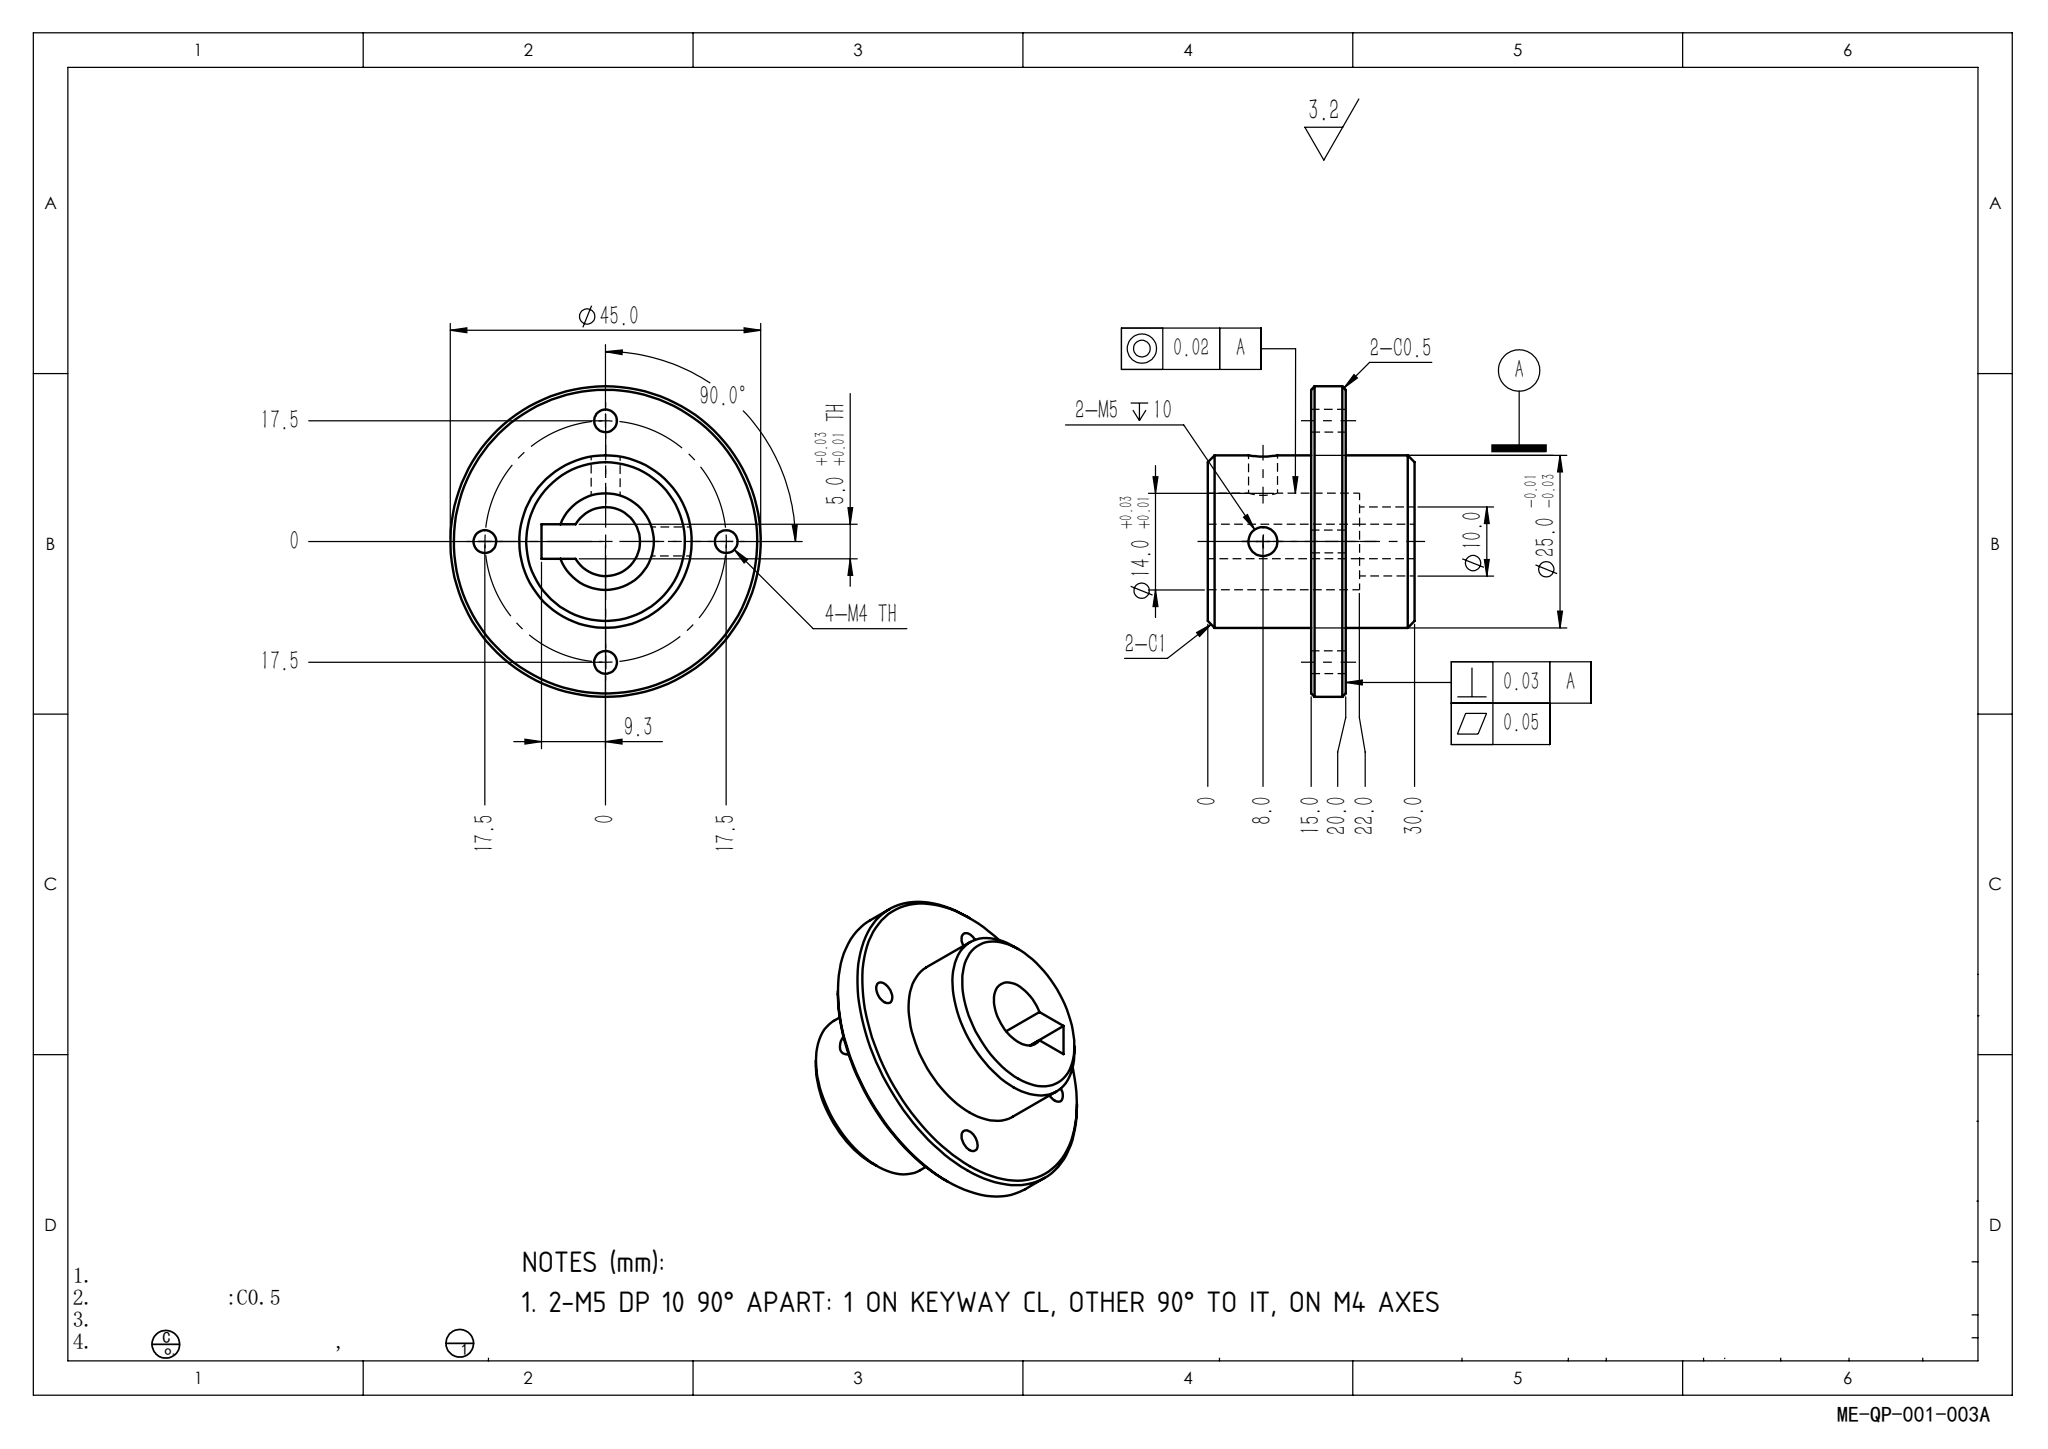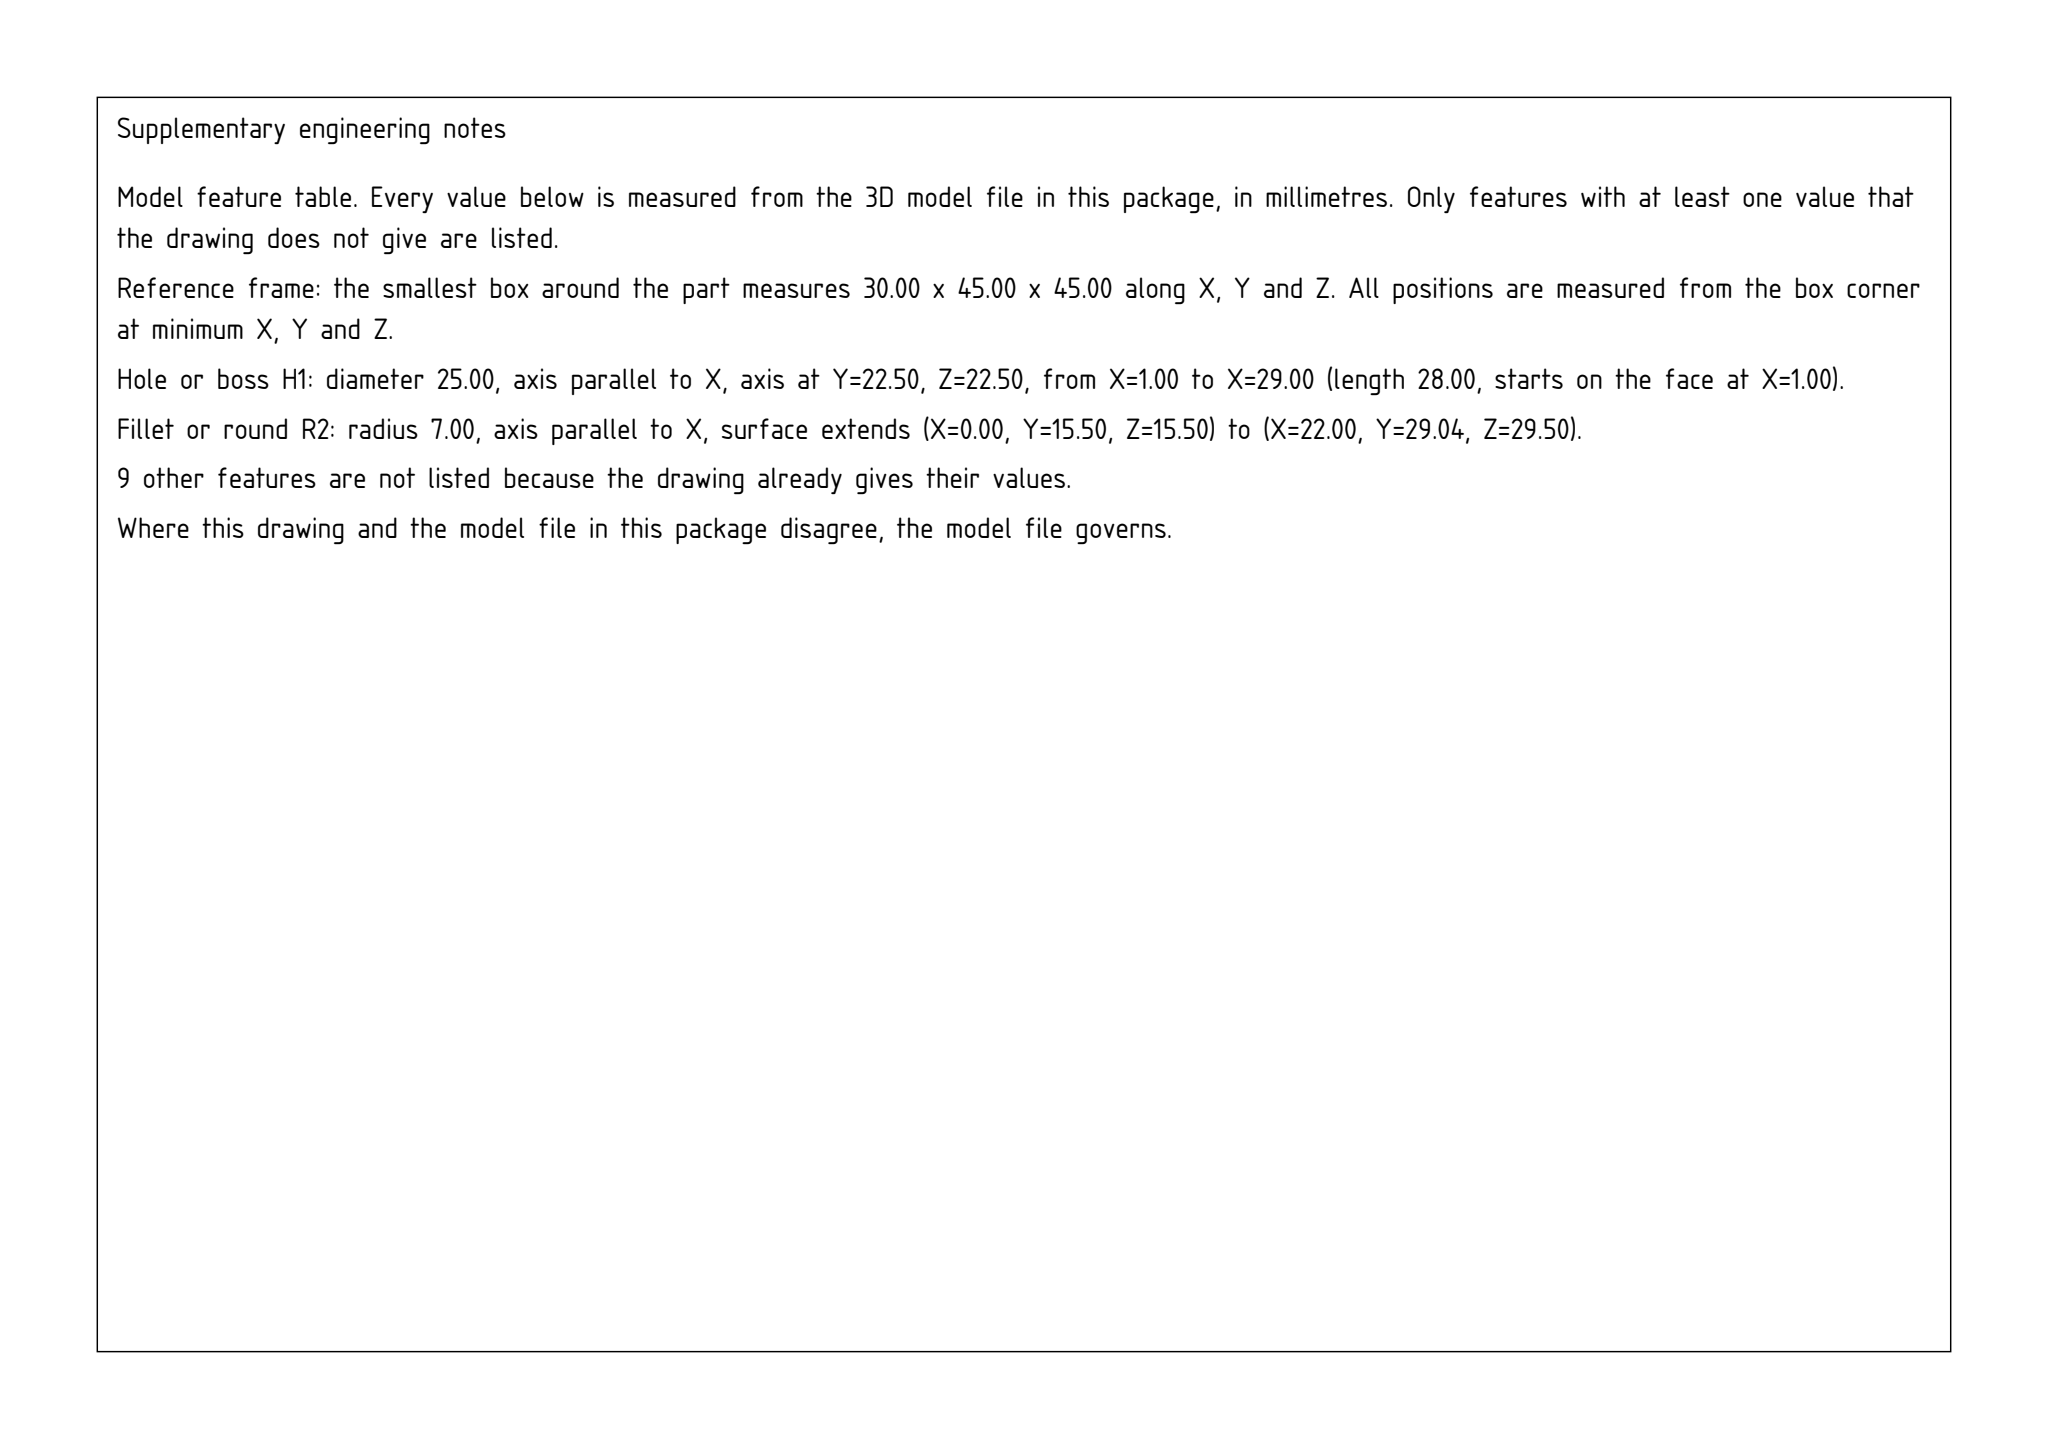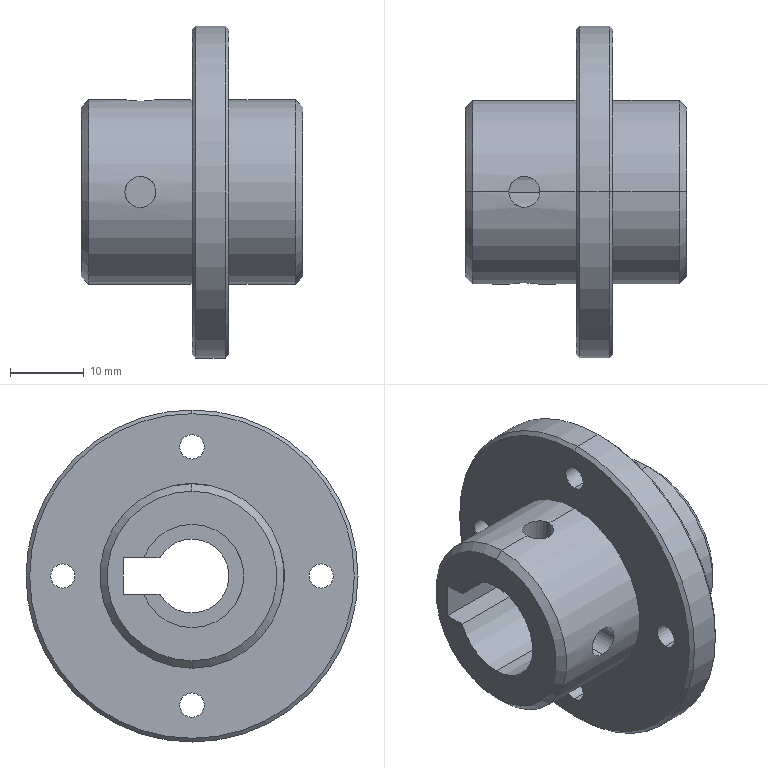Part | SolidWorks | mm | 1 solid | 40 faces | box 30 x 45 x 45 mm | volume 15323 mm3 | cylinder 24 | cone 8 | plane 8 | commonest cylinder face diameters 3.3 x8 4.2 x4 25 x4 10 x3 14 x3 45 x2
Drawing notes:
2-M5 DP 10 90° APART: 1 ON KEYWAY CL, OTHER 90° TO IT, ON M4 AXES | from the solid: Cyl 4.2 axis Y at (x=8, z=22.5) and cyl 4.2 axis Z at (x=8, y=22.5) -> axes perpendicular, both through part axis (22.5,22.5); keyway plane y=31.8 lies on +Y CL; 4x Ø3.3 at (5,22.5),(22.5,5),(22.5,40),(40,22.5) = same two axes
build123d program:
from build123d import *

# Parameters (mm, degrees)
SKETCH2_R               = 7
CUT_EXTRUDE1_DEPTH      = 22
SKETCH3_R               = 5
CUT_EXTRUDE2_DEPTH      = 44.732
SKETCH4_W               = 5
SKETCH4_H               = 8.882
CUT_EXTRUDE3_DEPTH      = 44.732
CUT_EXTRUDE4_REACH      = 37.178
SKETCH5_R               = 1.65
CIRPATTERN1_COUNT       = 4
CUT_EXTRUDE5_REACH      = 45.732
CUT_EXTRUDE5_END_RADIUS = 12.5
SKETCH6_R               = 2.1
CIRPATTERN2_COUNT       = 2
CIRPATTERN2_ANGLE       = 90
CHAMFER1_SIZE           = 1
CHAMFER2_SIZE           = 0.5


with BuildPart() as part:
    # Sketch1 → Revolve1 (revolve)
    with BuildSketch(Plane.XY, mode=Mode.PRIVATE) as revolve1_sk:
        Polygon((0, 0), (0, 12.5), (-10, 12.5), (-10, 22.5), (-15, 22.5), (-15, 12.5), (-30, 12.5), (-30, 0), align=None)
    revolve(revolve1_sk.sketch.rotate(Axis((0, 0, 0), (-1, 0, 0)), 90), axis=Axis((0, 0, 0), (-1, 0, 0)))

    # Sketch2 → Cut-Extrude1 (cut)
    with BuildSketch(Plane.ZY.offset(30)):
        Circle(SKETCH2_R)
    extrude(amount=-CUT_EXTRUDE1_DEPTH, mode=Mode.SUBTRACT)

    # Sketch3 → Cut-Extrude2 (cut, through all)
    with BuildSketch(Plane(origin=(0, 0, 0), x_dir=(0, 0, -1), z_dir=(1, 0, 0))):
        Circle(SKETCH3_R)
    extrude(amount=-CUT_EXTRUDE2_DEPTH, mode=Mode.SUBTRACT)

    # Sketch4 → Cut-Extrude3 (cut, through all)
    with BuildSketch(Plane(origin=(0, 0, 0), x_dir=(0, 0, -1), z_dir=(1, 0, 0))):
        with Locations((0, 4.859)):
            Rectangle(SKETCH4_W, SKETCH4_H)
    extrude(amount=-CUT_EXTRUDE3_DEPTH, mode=Mode.SUBTRACT)

    # Sketch5 → Cut-Extrude4 (cut, up to next)
    with BuildSketch(Plane.ZY.offset(15), mode=Mode.PRIVATE) as cut_extrude4_sk1:
        with Locations((0, 17.5)):
            Circle(SKETCH5_R)
    cut_extrude4_tool1 = extrude(cut_extrude4_sk1.sketch, amount=-CUT_EXTRUDE4_REACH, mode=Mode.PRIVATE) & part.part
    cut_extrude4 = cut_extrude4_tool1.solids().sort_by_distance((-15, 17.5, 0))[0]
    add(cut_extrude4, mode=Mode.SUBTRACT)

    # CirPattern1: Cut-Extrude4 ×4 about axis
    cirpattern1_axis = Axis((0, 0, 0), (1, 0, 0))
    for i in range(1, CIRPATTERN1_COUNT):
        add(cut_extrude4.rotate(cirpattern1_axis, i * 360 / CIRPATTERN1_COUNT), mode=Mode.SUBTRACT)

    # Cut-Extrude5: up to this cylinder (the profile starts inside it)
    cut_extrude5_end = Plane(origin=(-22, 0, 0), z_dir=(1, 0, 0)) * Cylinder(CUT_EXTRUDE5_END_RADIUS, 117.464, mode=Mode.PRIVATE)
    # Sketch6 → Cut-Extrude5 (cut, up to the surface)
    with BuildSketch(Plane.XY, mode=Mode.PRIVATE) as cut_extrude5_sk1:
        with Locations(Location((-22, 0, 0), (0, 0, 180))):
            Circle(SKETCH6_R)
    cut_extrude5_tool1 = extrude(cut_extrude5_sk1.sketch, amount=CUT_EXTRUDE5_REACH, mode=Mode.PRIVATE) & cut_extrude5_end
    cut_extrude5 = cut_extrude5_tool1.solids().sort_by_distance((-22, 0, 0))[0]
    add(cut_extrude5, mode=Mode.SUBTRACT)

    # CirPattern2: Cut-Extrude5 ×2 about axis
    cirpattern2_axis = Axis((-15, 0, 0), (1, 0, 0))
    for i in range(1, CIRPATTERN2_COUNT):
        add(cut_extrude5.rotate(cirpattern2_axis, i * CIRPATTERN2_ANGLE / (CIRPATTERN2_COUNT - 1)), mode=Mode.SUBTRACT)

    # Chamfer1
    chamfer1_edges = [part.edges().sort_by_distance(p)[0] for p in [
        (-30, 0, 12.5),
        (0, 0, 12.5),
    ]]
    chamfer(chamfer1_edges, length=CHAMFER1_SIZE)

    # Chamfer2
    chamfer2_edges = [part.edges().sort_by_distance(p)[0] for p in [
        (-15, 0, 22.5),
        (-10, 0, 22.5),
    ]]
    chamfer(chamfer2_edges, length=CHAMFER2_SIZE)


solid = part.part